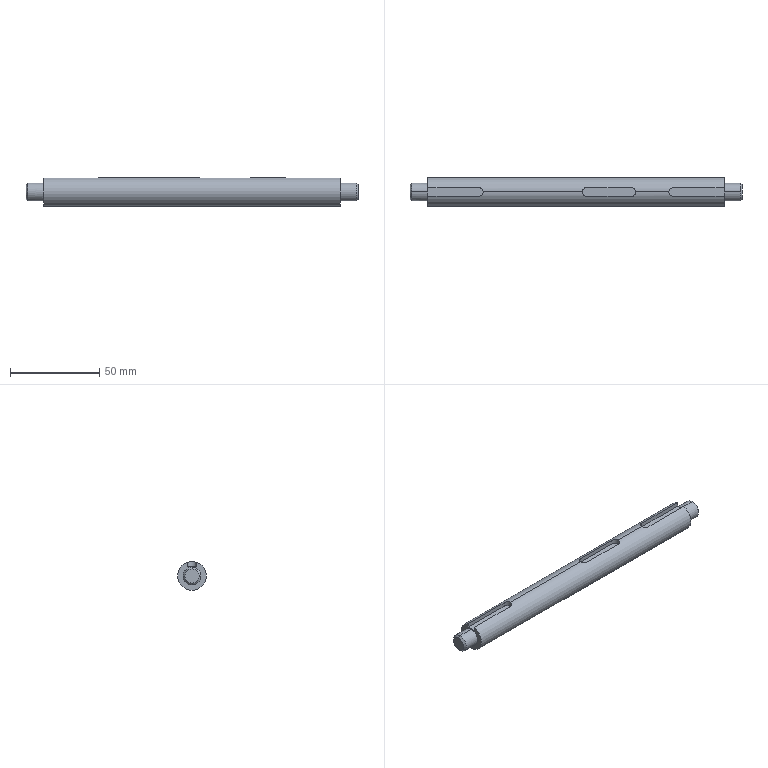CAM job | Mastercam | mm | 5 operations | part box 186 x 16 x 16
1. Contour (Ramp) | 7 - 4 平铣刀
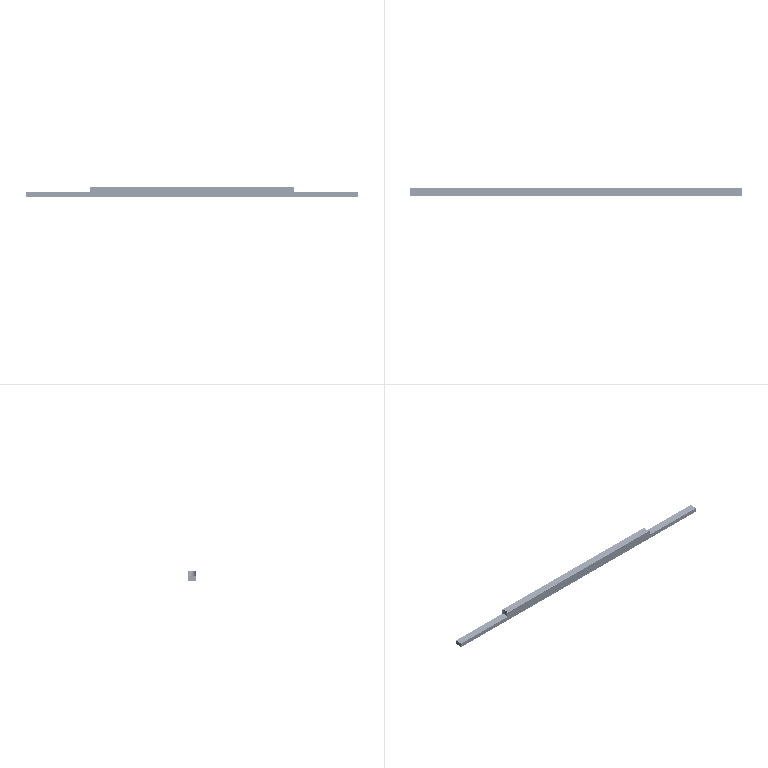2. Contour (Ramp) | 7 - 4 平铣刀
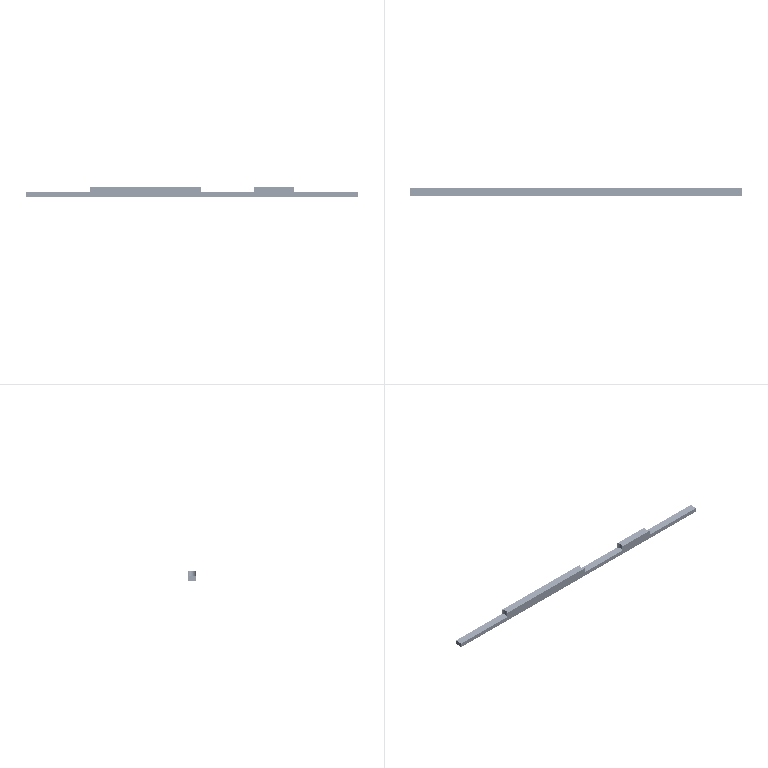3. Contour (2D) | 8 - 4 平铣刀
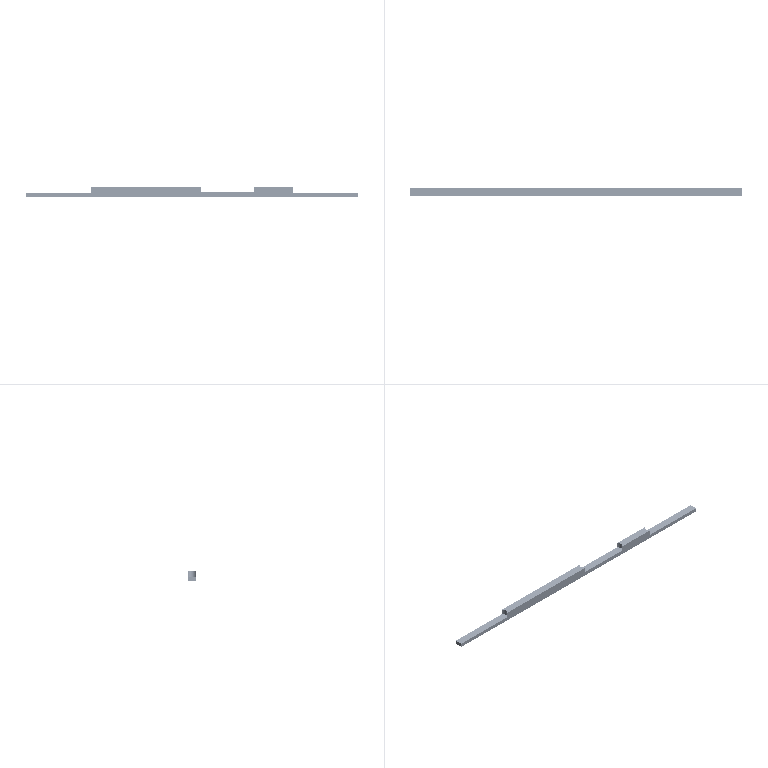4. Contour (2D) | 8 - 4 平铣刀
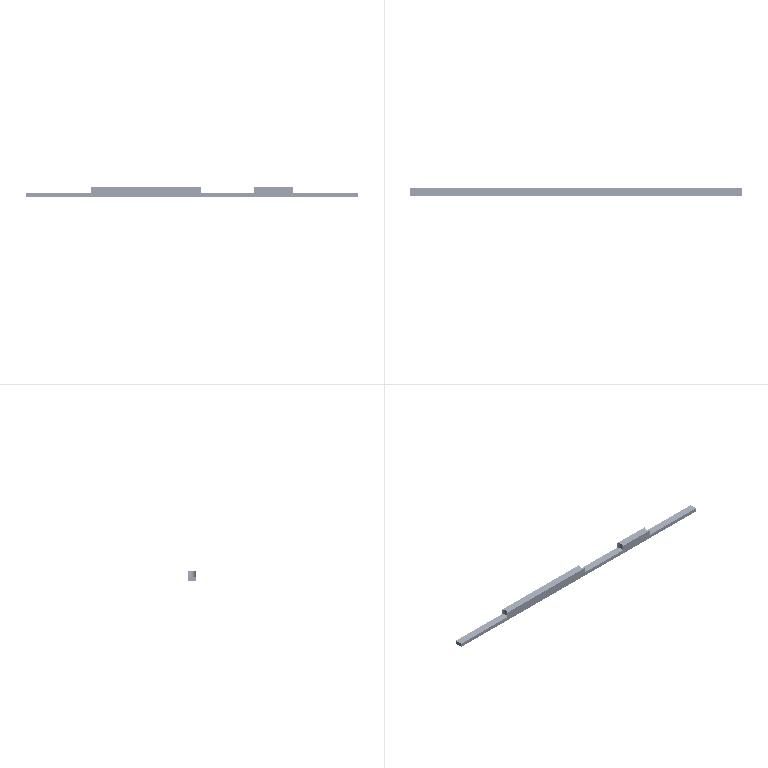5. Contour (3D chamfer) | 3 - 4 倒角刀